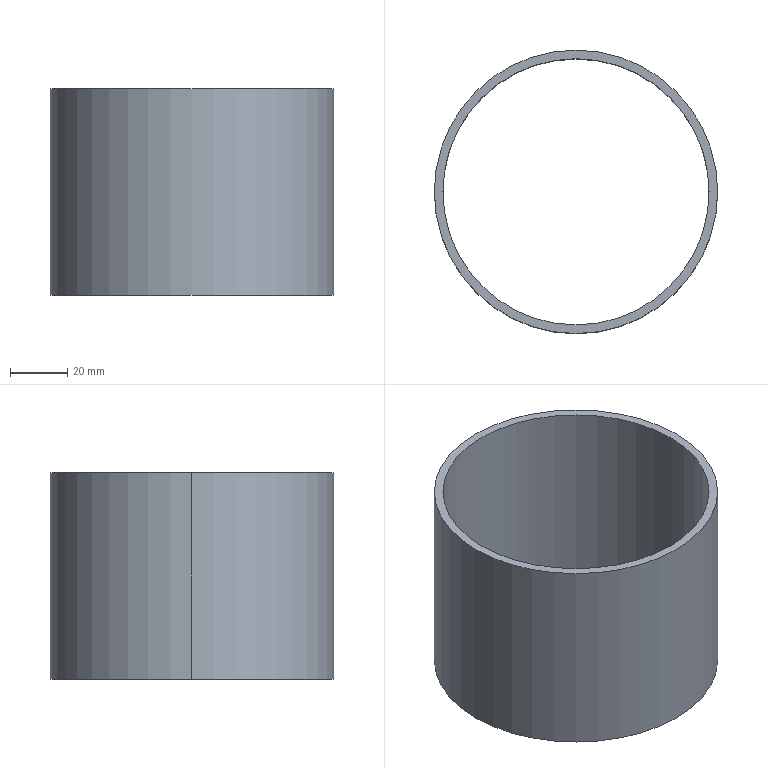Component | SolidWorks | Workpiece-1 | 1 solid | 6 faces | box 98.91 x 98.91 x 72 mm | volume 65082 mm3 | cylinder 4 | plane 2 | commonest cylinder face diameters 92.909 x2 98.909 x2
build123d program:
from build123d import *

# Parameters (mm, degrees)
SKETCH1_R           = 49.455
SKETCH1_R_2         = 46.455
EXTRUDE_THIN1_DEPTH = 72


with BuildPart() as part:
    # Sketch1 → Extrude-Thin1 (new body)
    with BuildSketch(Plane.XY):
        Circle(SKETCH1_R)
        Circle(SKETCH1_R_2, mode=Mode.SUBTRACT)
    extrude(amount=EXTRUDE_THIN1_DEPTH)


solid = part.part

# Placed as in the assembly
solid = solid.moved(Location((0, 0, -90), (0, 0, 0)))
STEP:
#1=COLOUR_RGB('',0.7922,0.8196,0.9333);
#2=FILL_AREA_STYLE_COLOUR('',#1);
#3=FILL_AREA_STYLE('',(#2));
#4=SURFACE_STYLE_FILL_AREA(#3);
#5=SURFACE_SIDE_STYLE('',(#4));
#6=SURFACE_STYLE_USAGE(.BOTH.,#5);
#7=PRESENTATION_STYLE_ASSIGNMENT((#6));
#8=CARTESIAN_POINT('',(1.829,0.,-3.543));
#9=VERTEX_POINT('',#8);
#10=CARTESIAN_POINT('',(-1.829,0.,-3.543));
#11=VERTEX_POINT('',#10);
#12=CARTESIAN_POINT('',(0.,0.,-3.543));
#13=DIRECTION('',(0.,0.,-1.));
#14=DIRECTION('',(-1.,0.,0.));
#15=AXIS2_PLACEMENT_3D('',#12,#13,#14);
#16=CIRCLE('',#15,1.829);
#17=EDGE_CURVE('',#9,#11,#16,.T.);
#18=ORIENTED_EDGE('',*,*,#17,.T.);
#19=CARTESIAN_POINT('',(-1.829,0.,-0.7087));
#20=VERTEX_POINT('',#19);
#21=CARTESIAN_POINT('',(-1.829,0.,-3.543));
#22=DIRECTION('',(0.,0.,1.));
#23=VECTOR('',#22,39.37);
#24=LINE('',#21,#23);
#25=EDGE_CURVE('',#11,#20,#24,.T.);
#26=ORIENTED_EDGE('',*,*,#25,.T.);
#27=CARTESIAN_POINT('',(1.829,0.,-0.7087));
#28=VERTEX_POINT('',#27);
#29=CARTESIAN_POINT('',(0.,0.,-0.7087));
#30=DIRECTION('',(0.,0.,-1.));
#31=DIRECTION('',(-1.,0.,0.));
#32=AXIS2_PLACEMENT_3D('',#29,#30,#31);
#33=CIRCLE('',#32,1.829);
#34=EDGE_CURVE('',#28,#20,#33,.T.);
#35=ORIENTED_EDGE('',*,*,#34,.F.);
#36=CARTESIAN_POINT('',(1.829,0.,-3.543));
#37=DIRECTION('',(0.,0.,1.));
#38=VECTOR('',#37,39.37);
#39=LINE('',#36,#38);
#40=EDGE_CURVE('',#9,#28,#39,.T.);
#41=ORIENTED_EDGE('',*,*,#40,.F.);
#42=EDGE_LOOP('',(#18,#26,#35,#41));
#43=FACE_OUTER_BOUND('',#42,.T.);
#44=CARTESIAN_POINT('',(0.,0.,-3.543));
#45=DIRECTION('',(0.,0.,1.));
#46=DIRECTION('',(1.,0.,0.));
#47=AXIS2_PLACEMENT_3D('',#44,#45,#46);
#48=CYLINDRICAL_SURFACE('',#47,1.829);
#49=ADVANCED_FACE('',(#43),#48,.F.);
#50=CARTESIAN_POINT('',(-1.947,0.,-3.543));
#51=VERTEX_POINT('',#50);
#52=CARTESIAN_POINT('',(1.947,0.,-3.543));
#53=VERTEX_POINT('',#52);
#54=CARTESIAN_POINT('',(0.,0.,-3.543));
#55=DIRECTION('',(0.,0.,-1.));
#56=DIRECTION('',(-1.,0.,0.));
#57=AXIS2_PLACEMENT_3D('',#54,#55,#56);
#58=CIRCLE('',#57,1.947);
#59=EDGE_CURVE('',#51,#53,#58,.T.);
#60=ORIENTED_EDGE('',*,*,#59,.F.);
#61=CARTESIAN_POINT('',(-1.947,0.,-0.7087));
#62=VERTEX_POINT('',#61);
#63=CARTESIAN_POINT('',(-1.947,0.,-3.543));
#64=DIRECTION('',(0.,0.,1.));
#65=VECTOR('',#64,39.37);
#66=LINE('',#63,#65);
#67=EDGE_CURVE('',#51,#62,#66,.T.);
#68=ORIENTED_EDGE('',*,*,#67,.T.);
#69=CARTESIAN_POINT('',(1.947,0.,-0.7087));
#70=VERTEX_POINT('',#69);
#71=CARTESIAN_POINT('',(0.,0.,-0.7087));
#72=DIRECTION('',(0.,0.,-1.));
#73=DIRECTION('',(-1.,0.,0.));
#74=AXIS2_PLACEMENT_3D('',#71,#72,#73);
#75=CIRCLE('',#74,1.947);
#76=EDGE_CURVE('',#62,#70,#75,.T.);
#77=ORIENTED_EDGE('',*,*,#76,.T.);
#78=CARTESIAN_POINT('',(1.947,0.,-3.543));
#79=DIRECTION('',(0.,0.,1.));
#80=VECTOR('',#79,39.37);
#81=LINE('',#78,#80);
#82=EDGE_CURVE('',#53,#70,#81,.T.);
#83=ORIENTED_EDGE('',*,*,#82,.F.);
#84=EDGE_LOOP('',(#60,#68,#77,#83));
#85=FACE_OUTER_BOUND('',#84,.T.);
#86=CARTESIAN_POINT('',(0.,0.,-3.543));
#87=DIRECTION('',(0.,0.,1.));
#88=DIRECTION('',(1.,0.,0.));
#89=AXIS2_PLACEMENT_3D('',#86,#87,#88);
#90=CYLINDRICAL_SURFACE('',#89,1.947);
#91=ADVANCED_FACE('',(#85),#90,.T.);
#92=CARTESIAN_POINT('',(0.,0.,-3.543));
#93=DIRECTION('',(0.,0.,-1.));
#94=DIRECTION('',(-1.,0.,0.));
#95=AXIS2_PLACEMENT_3D('',#92,#93,#94);
#96=CIRCLE('',#95,1.947);
#97=EDGE_CURVE('',#53,#51,#96,.T.);
#98=ORIENTED_EDGE('',*,*,#97,.T.);
#99=ORIENTED_EDGE('',*,*,#59,.T.);
#100=EDGE_LOOP('',(#98,#99));
#101=FACE_OUTER_BOUND('',#100,.T.);
#102=ORIENTED_EDGE('',*,*,#17,.F.);
#103=CARTESIAN_POINT('',(0.,0.,-3.543));
#104=DIRECTION('',(0.,0.,-1.));
#105=DIRECTION('',(-1.,0.,0.));
#106=AXIS2_PLACEMENT_3D('',#103,#104,#105);
#107=CIRCLE('',#106,1.829);
#108=EDGE_CURVE('',#11,#9,#107,.T.);
#109=ORIENTED_EDGE('',*,*,#108,.F.);
#110=EDGE_LOOP('',(#102,#109));
#111=FACE_BOUND('',#110,.T.);
#112=CARTESIAN_POINT('',(0.,0.,-3.543));
#113=DIRECTION('',(0.,0.,-1.));
#114=DIRECTION('',(-1.,0.,0.));
#115=AXIS2_PLACEMENT_3D('',#112,#113,#114);
#116=PLANE('',#115);
#117=ADVANCED_FACE('',(#101,#111),#116,.T.);
#118=CARTESIAN_POINT('',(0.,0.,-0.7087));
#119=DIRECTION('',(0.,0.,-1.));
#120=DIRECTION('',(-1.,0.,0.));
#121=AXIS2_PLACEMENT_3D('',#118,#119,#120);
#122=CIRCLE('',#121,1.947);
#123=EDGE_CURVE('',#70,#62,#122,.T.);
#124=ORIENTED_EDGE('',*,*,#123,.F.);
#125=ORIENTED_EDGE('',*,*,#76,.F.);
#126=EDGE_LOOP('',(#124,#125));
#127=FACE_OUTER_BOUND('',#126,.T.);
#128=ORIENTED_EDGE('',*,*,#34,.T.);
#129=CARTESIAN_POINT('',(0.,0.,-0.7087));
#130=DIRECTION('',(0.,0.,-1.));
#131=DIRECTION('',(-1.,0.,0.));
#132=AXIS2_PLACEMENT_3D('',#129,#130,#131);
#133=CIRCLE('',#132,1.829);
#134=EDGE_CURVE('',#20,#28,#133,.T.);
#135=ORIENTED_EDGE('',*,*,#134,.T.);
#136=EDGE_LOOP('',(#128,#135));
#137=FACE_BOUND('',#136,.T.);
#138=CARTESIAN_POINT('',(0.,0.,-0.7087));
#139=DIRECTION('',(0.,0.,-1.));
#140=DIRECTION('',(-1.,0.,0.));
#141=AXIS2_PLACEMENT_3D('',#138,#139,#140);
#142=PLANE('',#141);
#143=ADVANCED_FACE('',(#127,#137),#142,.F.);
#144=ORIENTED_EDGE('',*,*,#67,.F.);
#145=ORIENTED_EDGE('',*,*,#97,.F.);
#146=ORIENTED_EDGE('',*,*,#82,.T.);
#147=ORIENTED_EDGE('',*,*,#123,.T.);
#148=EDGE_LOOP('',(#144,#145,#146,#147));
#149=FACE_OUTER_BOUND('',#148,.T.);
#150=CARTESIAN_POINT('',(0.,0.,-3.543));
#151=DIRECTION('',(0.,0.,1.));
#152=DIRECTION('',(1.,0.,0.));
#153=AXIS2_PLACEMENT_3D('',#150,#151,#152);
#154=CYLINDRICAL_SURFACE('',#153,1.947);
#155=ADVANCED_FACE('',(#149),#154,.T.);
#156=ORIENTED_EDGE('',*,*,#25,.F.);
#157=ORIENTED_EDGE('',*,*,#108,.T.);
#158=ORIENTED_EDGE('',*,*,#40,.T.);
#159=ORIENTED_EDGE('',*,*,#134,.F.);
#160=EDGE_LOOP('',(#156,#157,#158,#159));
#161=FACE_OUTER_BOUND('',#160,.T.);
#162=CARTESIAN_POINT('',(0.,0.,-3.543));
#163=DIRECTION('',(0.,0.,1.));
#164=DIRECTION('',(1.,0.,0.));
#165=AXIS2_PLACEMENT_3D('',#162,#163,#164);
#166=CYLINDRICAL_SURFACE('',#165,1.829);
#167=ADVANCED_FACE('',(#161),#166,.F.);
#168=CLOSED_SHELL('',(#49,#91,#117,#143,#155,#167));
#169=MANIFOLD_SOLID_BREP('',#168);
#170=STYLED_ITEM('',(#7),#169);
#171=PRESENTATION_LAYER_ASSIGNMENT('','',(#170));
#172=(LENGTH_UNIT()NAMED_UNIT(*)SI_UNIT($,.METRE.));
#173=LENGTH_MEASURE_WITH_UNIT(LENGTH_MEASURE(0.0254),#172);
#174=DIMENSIONAL_EXPONENTS(1.,0.,0.,0.,0.,0.,0.);
#175=(CONVERSION_BASED_UNIT('',#173)LENGTH_UNIT()NAMED_UNIT(#174));
#176=UNCERTAINTY_MEASURE_WITH_UNIT(LENGTH_MEASURE(0.00001),#175,'','');
#177=(NAMED_UNIT(*)PLANE_ANGLE_UNIT()SI_UNIT($,.RADIAN.));
#178=(NAMED_UNIT(*)SI_UNIT($,.STERADIAN.)SOLID_ANGLE_UNIT());
#179=(GEOMETRIC_REPRESENTATION_CONTEXT(3)GLOBAL_UNCERTAINTY_ASSIGNED_CONTEXT((#176))GLOBAL_UNIT_ASSIGNED_CONTEXT((#175,#177,#178))REPRESENTATION_CONTEXT('',''));
#180=MECHANICAL_DESIGN_GEOMETRIC_PRESENTATION_REPRESENTATION('',(#170),#179);
#181=CARTESIAN_POINT('',(0.,0.,0.));
#182=DIRECTION('',(0.,0.,1.));
#183=DIRECTION('',(1.,0.,0.));
#184=AXIS2_PLACEMENT_3D('',#181,#182,#183);
#185=(LENGTH_UNIT()NAMED_UNIT(*)SI_UNIT($,.METRE.));
#186=LENGTH_MEASURE_WITH_UNIT(LENGTH_MEASURE(0.0254),#185);
#187=DIMENSIONAL_EXPONENTS(1.,0.,0.,0.,0.,0.,0.);
#188=(CONVERSION_BASED_UNIT('',#186)LENGTH_UNIT()NAMED_UNIT(#187));
#189=UNCERTAINTY_MEASURE_WITH_UNIT(LENGTH_MEASURE(0.00001),#188,'','');
#190=(NAMED_UNIT(*)PLANE_ANGLE_UNIT()SI_UNIT($,.RADIAN.));
#191=(NAMED_UNIT(*)SI_UNIT($,.STERADIAN.)SOLID_ANGLE_UNIT());
#192=(GEOMETRIC_REPRESENTATION_CONTEXT(3)GLOBAL_UNCERTAINTY_ASSIGNED_CONTEXT((#189))GLOBAL_UNIT_ASSIGNED_CONTEXT((#188,#190,#191))REPRESENTATION_CONTEXT('',''));
#193=ADVANCED_BREP_SHAPE_REPRESENTATION('',(#169,#184),#192);